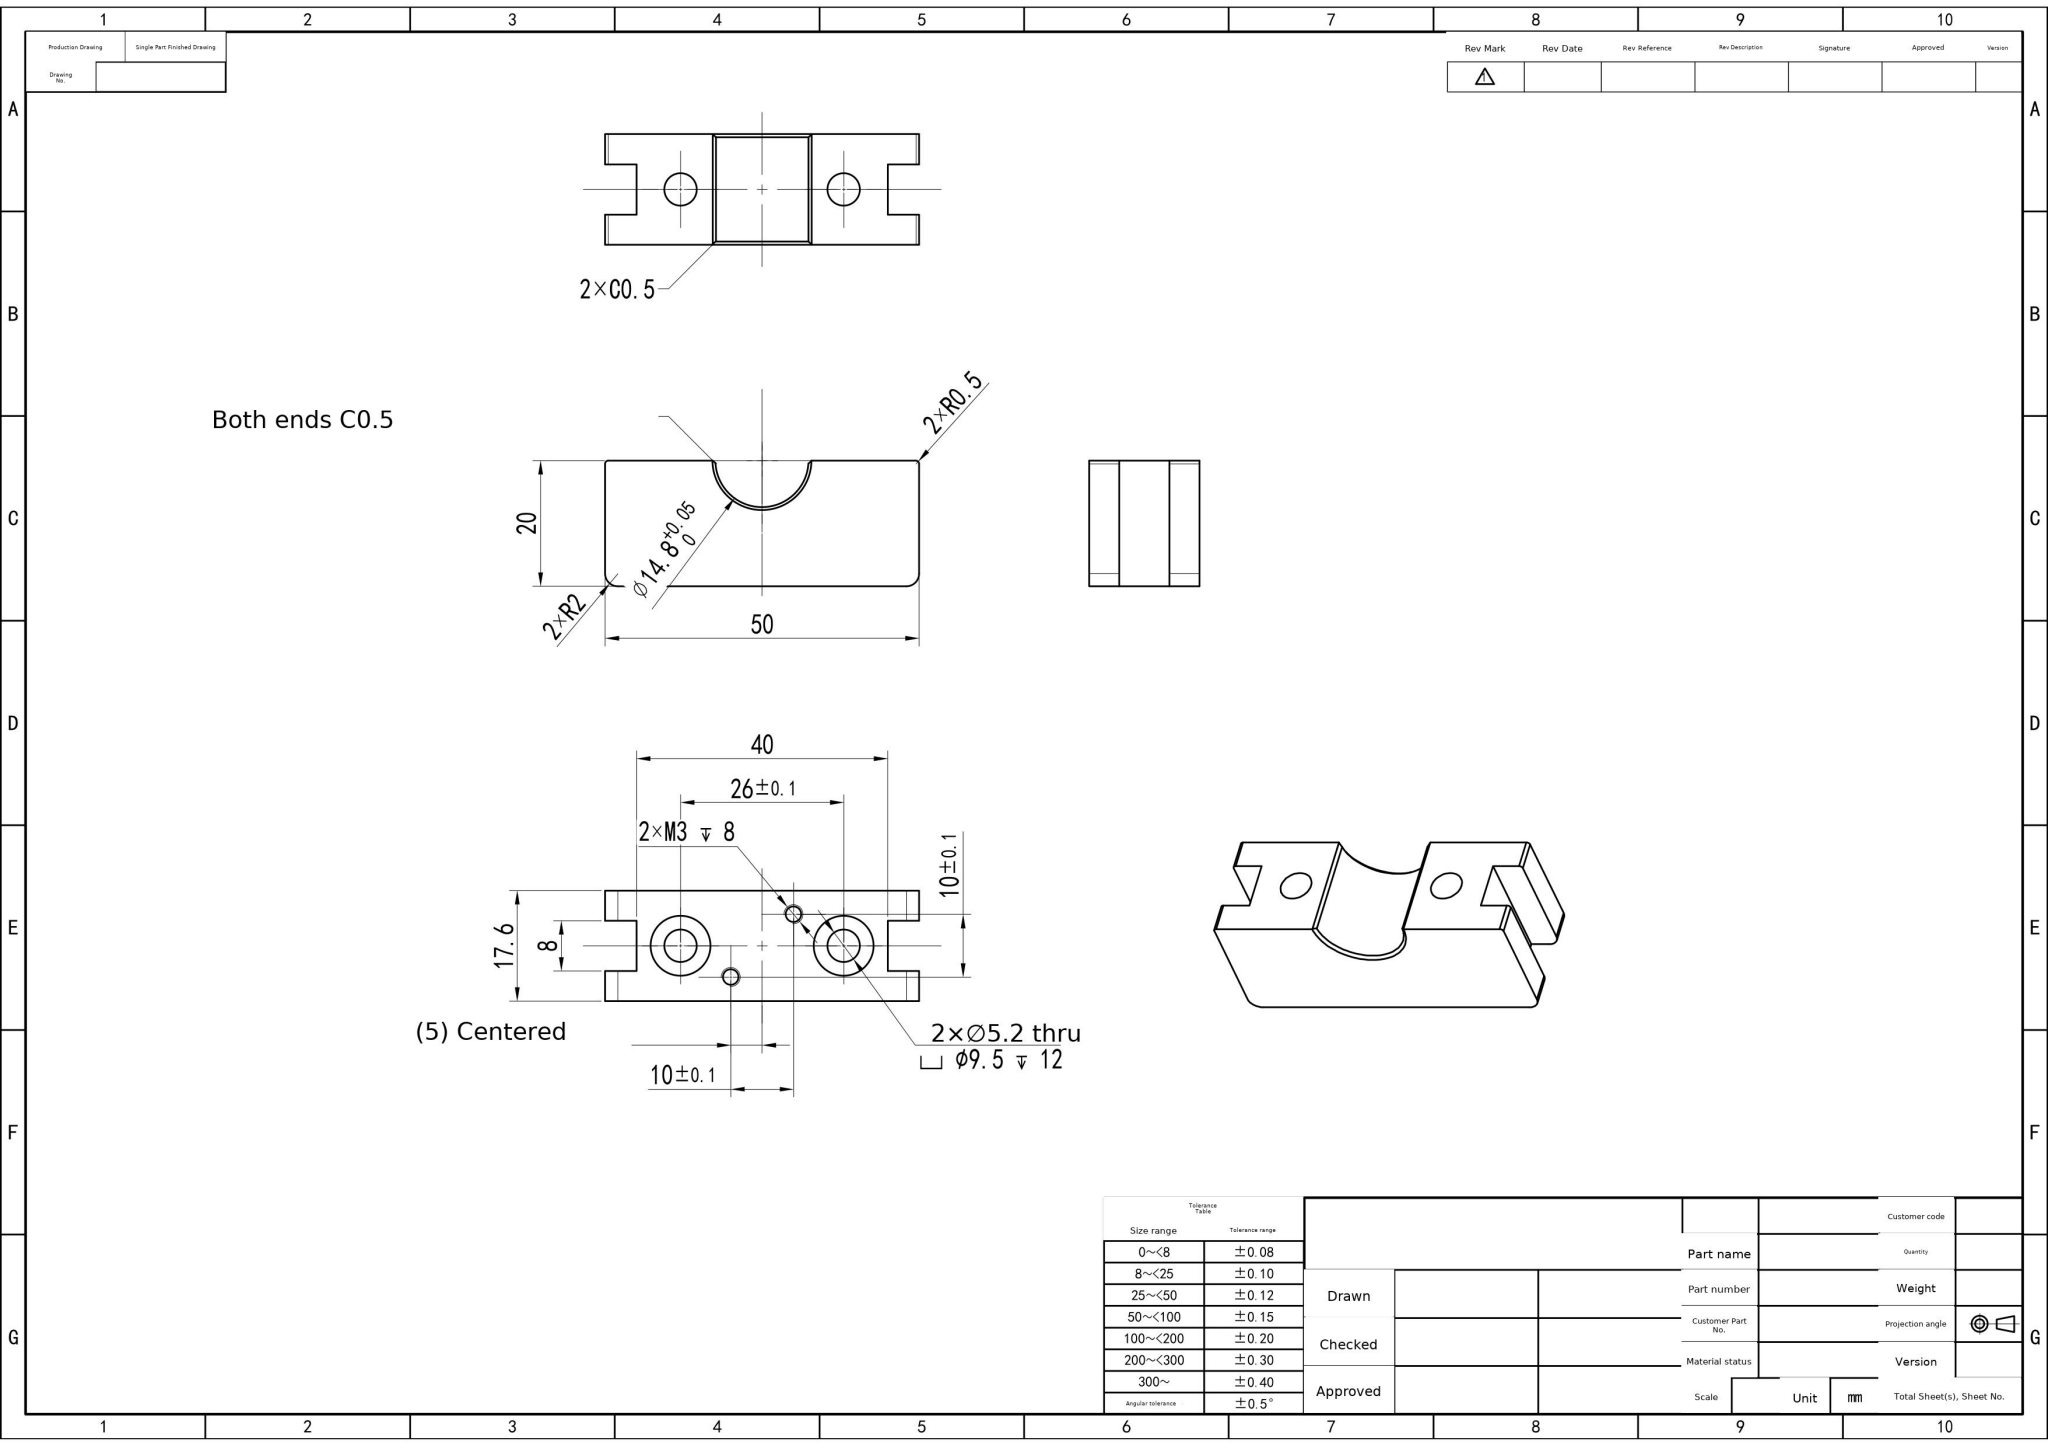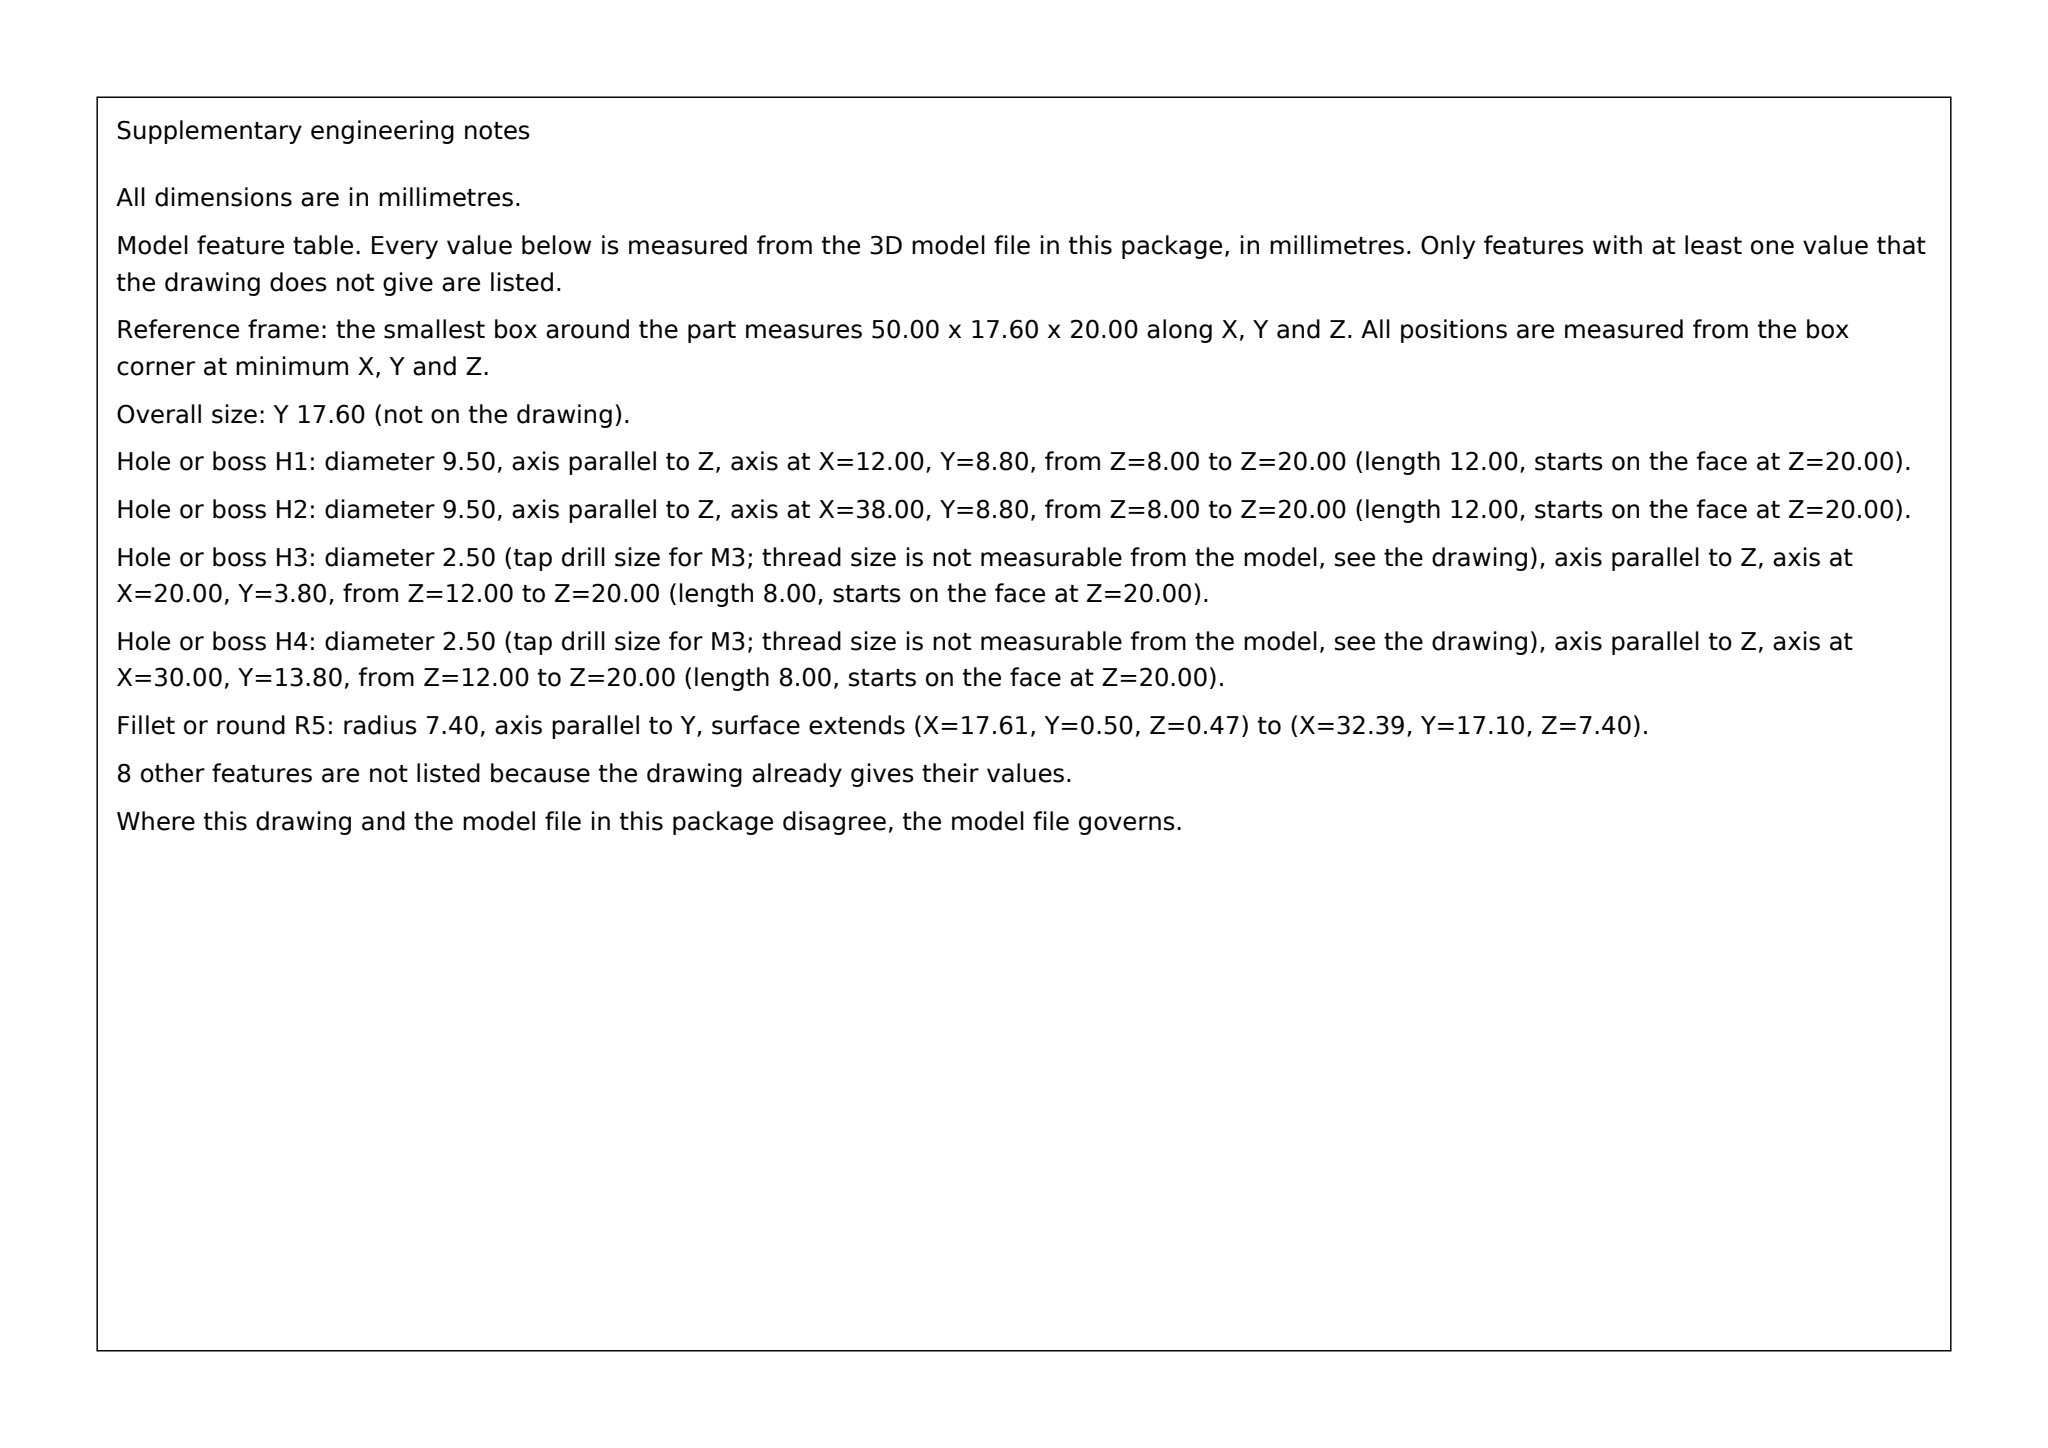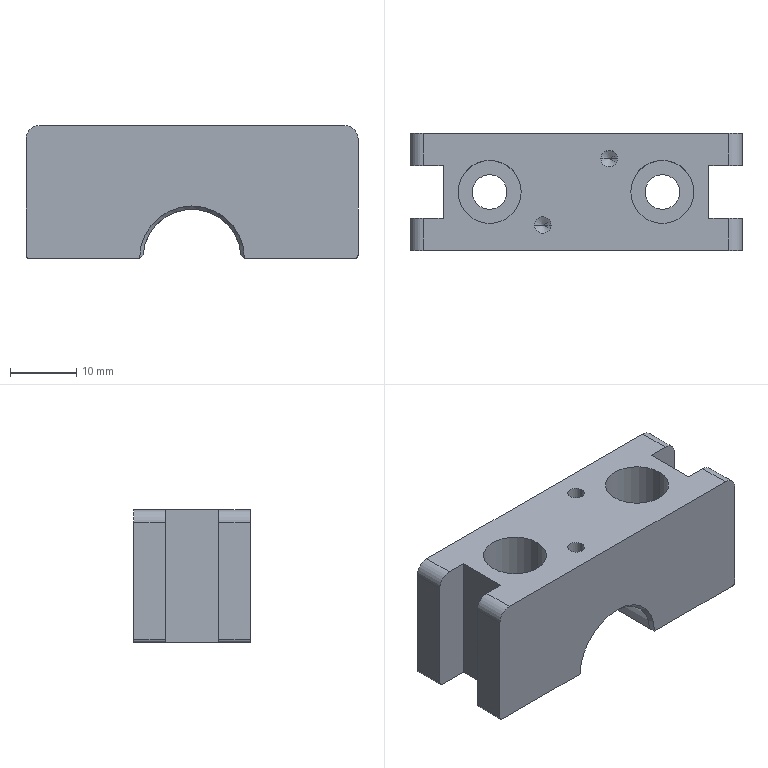Part | SolidWorks | mm | 1 solid | 47 faces | box 50 x 17.6 x 20 mm | volume 12337 mm3 | cylinder 21 | plane 19 | cone 7 | commonest cylinder face diameters 2.5 x4 9.5 x4 5.2 x4 4 x4 1 x4 14.8 x1